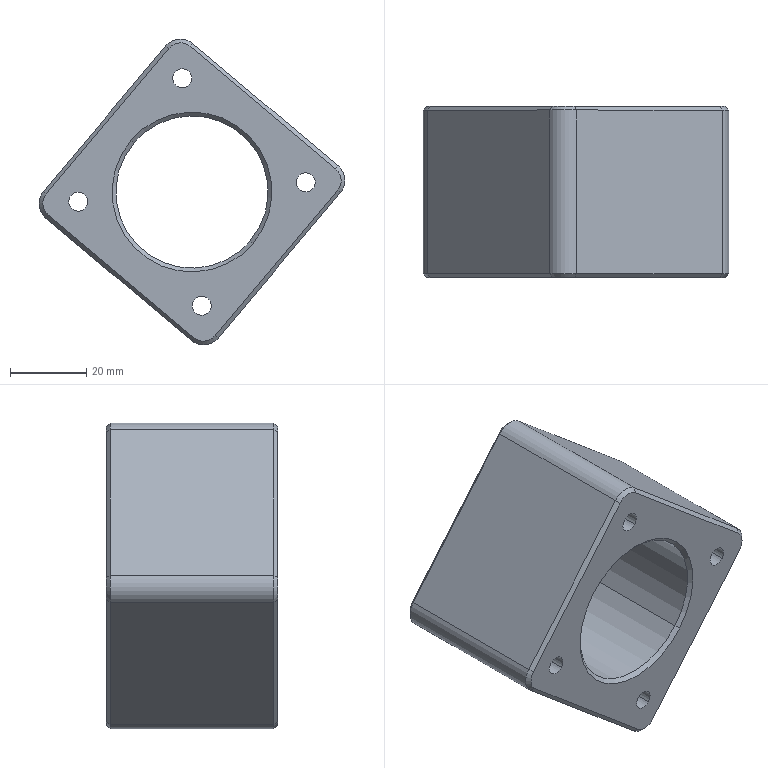Component | SolidWorks | 03LocatingBlock-1 | 1 solid | 40 faces | volume 100594 mm3 | cylinder 14 | plane 14 | cone 12 | commonest cylinder face diameters 5 x8 10 x4 40 x2 | material Aviation Aluminum-7075